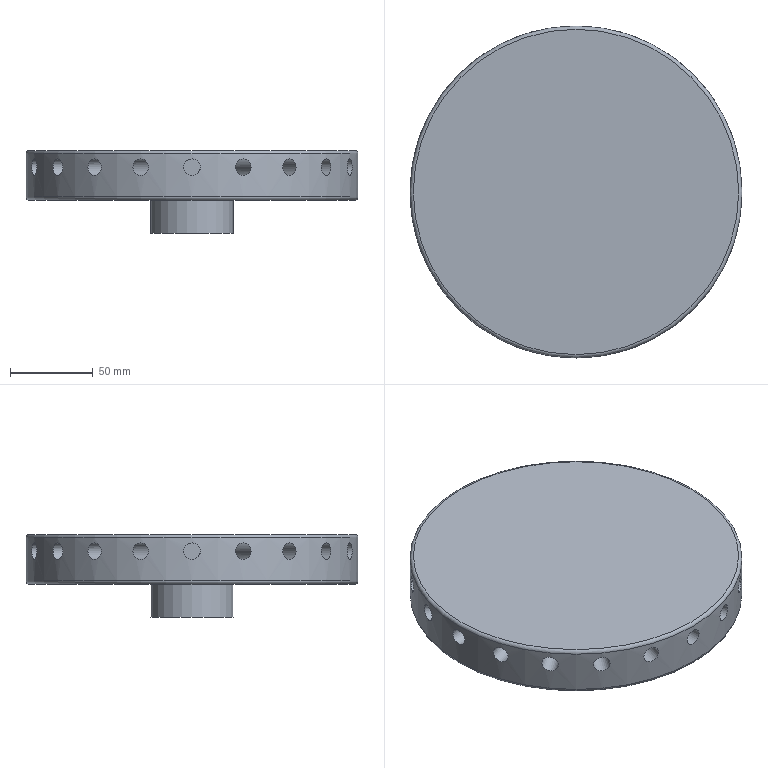Component | NX | ALT | 1 solid | 47 faces | volume 886485 mm3 | plane 23 | cylinder 22 | torus 2 | commonest cylinder face diameters 10 x20 200 x1 50 x1